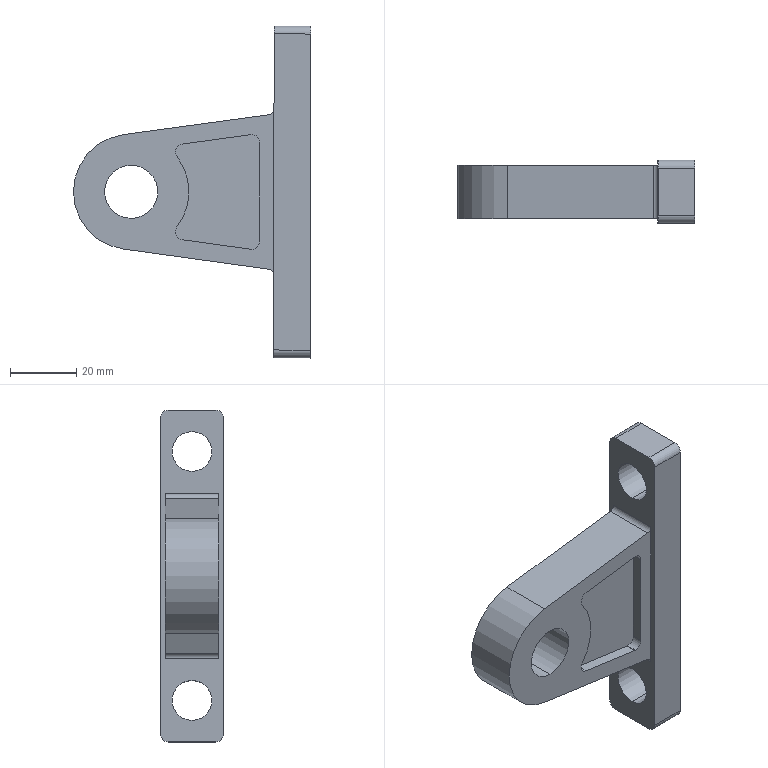Component | SolidWorks | RobotArmTelescopicCylinderSC32x500-1_MiddleEarFixingBlock1-1 | 1 solid | 43 faces | box 71.45 x 19 x 100.01 mm | volume 46285 mm3 | cylinder 25 | plane 18 | commonest cylinder face diameters 4.8 x14 12 x4 34.8 x3 16 x2 3.2 x2